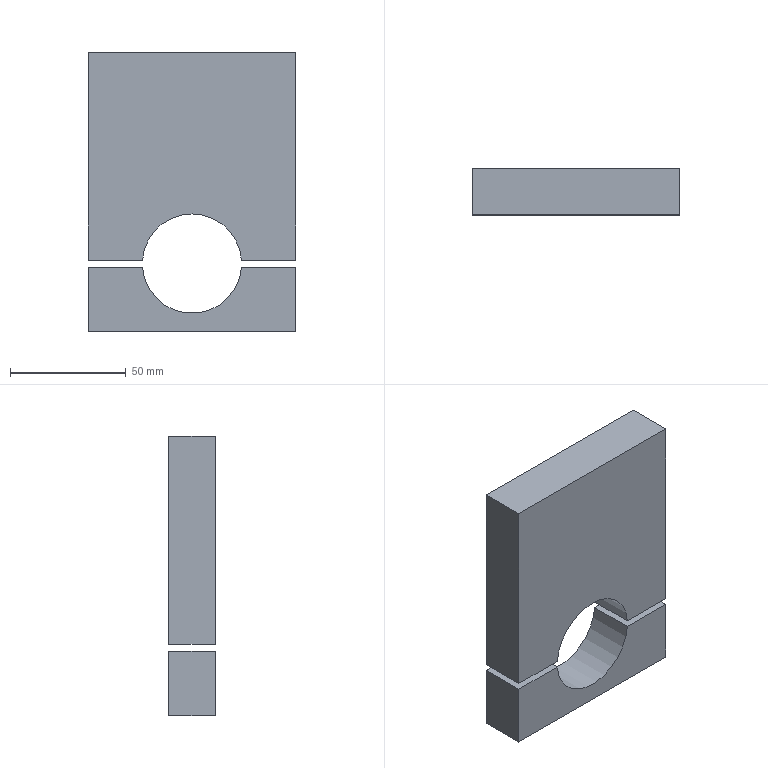Component | SolidWorks | YC1-250-04BalancerAssembly#16673-1_YC1-250-04-12#16673PipeSeat-1 | 2 solids | 29 faces | box 90 x 20 x 121 mm | volume 177905 mm3 | plane 14 | cylinder 11 | cone 4 | commonest cylinder face diameters 8.5 x4 11 x4 43 x3 | material Plain Carbon Steel
STEP:
#1=COLOUR_RGB('',0.7922,0.8196,0.9333);
#2=FILL_AREA_STYLE_COLOUR('',#1);
#3=FILL_AREA_STYLE('',(#2));
#4=SURFACE_STYLE_FILL_AREA(#3);
#5=SURFACE_SIDE_STYLE('',(#4));
#6=SURFACE_STYLE_USAGE(.BOTH.,#5);
#7=PRESENTATION_STYLE_ASSIGNMENT((#6));
#8=CARTESIAN_POINT('',(-16.929,179.528,-9.567));
#9=VERTEX_POINT('',#8);
#10=CARTESIAN_POINT('',(-16.496,179.528,-9.567));
#11=VERTEX_POINT('',#10);
#12=CARTESIAN_POINT('',(-16.713,179.528,-9.567));
#13=DIRECTION('',(0.,0.,1.));
#14=DIRECTION('',(-1.,0.,0.));
#15=AXIS2_PLACEMENT_3D('',#12,#13,#14);
#16=CIRCLE('',#15,0.2165);
#17=EDGE_CURVE('',#9,#11,#16,.T.);
#18=ORIENTED_EDGE('',*,*,#17,.T.);
#19=CARTESIAN_POINT('',(-16.496,179.528,-10.669));
#20=VERTEX_POINT('',#19);
#21=CARTESIAN_POINT('',(-16.496,179.528,-10.669));
#22=DIRECTION('',(0.,0.,-1.));
#23=VECTOR('',#22,39.37);
#24=LINE('',#21,#23);
#25=EDGE_CURVE('',#11,#20,#24,.T.);
#26=ORIENTED_EDGE('',*,*,#25,.T.);
#27=CARTESIAN_POINT('',(-16.929,179.528,-10.669));
#28=VERTEX_POINT('',#27);
#29=CARTESIAN_POINT('',(-16.713,179.528,-10.669));
#30=DIRECTION('',(0.,0.,-1.));
#31=DIRECTION('',(-1.,0.,0.));
#32=AXIS2_PLACEMENT_3D('',#29,#30,#31);
#33=CIRCLE('',#32,0.2165);
#34=EDGE_CURVE('',#20,#28,#33,.T.);
#35=ORIENTED_EDGE('',*,*,#34,.T.);
#36=CARTESIAN_POINT('',(-16.929,179.528,-10.669));
#37=DIRECTION('',(0.,0.,-1.));
#38=VECTOR('',#37,39.37);
#39=LINE('',#36,#38);
#40=EDGE_CURVE('',#9,#28,#39,.T.);
#41=ORIENTED_EDGE('',*,*,#40,.F.);
#42=EDGE_LOOP('',(#18,#26,#35,#41));
#43=FACE_OUTER_BOUND('',#42,.T.);
#44=CARTESIAN_POINT('',(-16.713,179.528,-10.669));
#45=DIRECTION('',(0.,0.,-1.));
#46=DIRECTION('',(-1.,0.,0.));
#47=AXIS2_PLACEMENT_3D('',#44,#45,#46);
#48=CYLINDRICAL_SURFACE('',#47,0.2165);
#49=ADVANCED_FACE('',(#43),#48,.F.);
#50=CARTESIAN_POINT('',(-19.724,179.528,-9.567));
#51=VERTEX_POINT('',#50);
#52=CARTESIAN_POINT('',(-19.291,179.528,-9.567));
#53=VERTEX_POINT('',#52);
#54=CARTESIAN_POINT('',(-19.508,179.528,-9.567));
#55=DIRECTION('',(0.,0.,1.));
#56=DIRECTION('',(-1.,0.,0.));
#57=AXIS2_PLACEMENT_3D('',#54,#55,#56);
#58=CIRCLE('',#57,0.2165);
#59=EDGE_CURVE('',#51,#53,#58,.T.);
#60=ORIENTED_EDGE('',*,*,#59,.T.);
#61=CARTESIAN_POINT('',(-19.291,179.528,-10.669));
#62=VERTEX_POINT('',#61);
#63=CARTESIAN_POINT('',(-19.291,179.528,-10.669));
#64=DIRECTION('',(0.,0.,-1.));
#65=VECTOR('',#64,39.37);
#66=LINE('',#63,#65);
#67=EDGE_CURVE('',#53,#62,#66,.T.);
#68=ORIENTED_EDGE('',*,*,#67,.T.);
#69=CARTESIAN_POINT('',(-19.724,179.528,-10.669));
#70=VERTEX_POINT('',#69);
#71=CARTESIAN_POINT('',(-19.508,179.528,-10.669));
#72=DIRECTION('',(0.,0.,-1.));
#73=DIRECTION('',(-1.,0.,0.));
#74=AXIS2_PLACEMENT_3D('',#71,#72,#73);
#75=CIRCLE('',#74,0.2165);
#76=EDGE_CURVE('',#62,#70,#75,.T.);
#77=ORIENTED_EDGE('',*,*,#76,.T.);
#78=CARTESIAN_POINT('',(-19.724,179.528,-10.669));
#79=DIRECTION('',(0.,0.,-1.));
#80=VECTOR('',#79,39.37);
#81=LINE('',#78,#80);
#82=EDGE_CURVE('',#51,#70,#81,.T.);
#83=ORIENTED_EDGE('',*,*,#82,.F.);
#84=EDGE_LOOP('',(#60,#68,#77,#83));
#85=FACE_OUTER_BOUND('',#84,.T.);
#86=CARTESIAN_POINT('',(-19.508,179.528,-10.669));
#87=DIRECTION('',(0.,0.,-1.));
#88=DIRECTION('',(-1.,0.,0.));
#89=AXIS2_PLACEMENT_3D('',#86,#87,#88);
#90=CYLINDRICAL_SURFACE('',#89,0.2165);
#91=ADVANCED_FACE('',(#85),#90,.F.);
#92=CARTESIAN_POINT('',(-19.882,179.134,-9.567));
#93=VERTEX_POINT('',#92);
#94=CARTESIAN_POINT('',(-19.882,179.134,-10.669));
#95=VERTEX_POINT('',#94);
#96=CARTESIAN_POINT('',(-19.882,179.134,-9.508));
#97=DIRECTION('',(0.,0.,-1.));
#98=VECTOR('',#97,39.37);
#99=LINE('',#96,#98);
#100=EDGE_CURVE('',#93,#95,#99,.T.);
#101=ORIENTED_EDGE('',*,*,#100,.T.);
#102=CARTESIAN_POINT('',(-16.339,179.134,-10.669));
#103=VERTEX_POINT('',#102);
#104=CARTESIAN_POINT('',(-18.11,179.134,-10.669));
#105=DIRECTION('',(1.,0.,0.));
#106=VECTOR('',#105,39.37);
#107=LINE('',#104,#106);
#108=EDGE_CURVE('',#95,#103,#107,.T.);
#109=ORIENTED_EDGE('',*,*,#108,.T.);
#110=CARTESIAN_POINT('',(-16.339,179.134,-9.567));
#111=VERTEX_POINT('',#110);
#112=CARTESIAN_POINT('',(-16.339,179.134,-9.508));
#113=DIRECTION('',(0.,0.,1.));
#114=VECTOR('',#113,39.37);
#115=LINE('',#112,#114);
#116=EDGE_CURVE('',#103,#111,#115,.T.);
#117=ORIENTED_EDGE('',*,*,#116,.T.);
#118=CARTESIAN_POINT('',(-17.266,179.134,-9.567));
#119=VERTEX_POINT('',#118);
#120=CARTESIAN_POINT('',(-18.11,179.134,-9.567));
#121=DIRECTION('',(-1.,0.,0.));
#122=VECTOR('',#121,39.37);
#123=LINE('',#120,#122);
#124=EDGE_CURVE('',#111,#119,#123,.T.);
#125=ORIENTED_EDGE('',*,*,#124,.T.);
#126=CARTESIAN_POINT('',(-18.955,179.134,-9.567));
#127=VERTEX_POINT('',#126);
#128=CARTESIAN_POINT('',(-18.11,179.134,-9.508));
#129=DIRECTION('',(0.,1.,0.));
#130=DIRECTION('',(0.,0.,1.));
#131=AXIS2_PLACEMENT_3D('',#128,#129,#130);
#132=CIRCLE('',#131,0.8465);
#133=EDGE_CURVE('',#119,#127,#132,.T.);
#134=ORIENTED_EDGE('',*,*,#133,.T.);
#135=CARTESIAN_POINT('',(-18.11,179.134,-9.567));
#136=DIRECTION('',(-1.,0.,0.));
#137=VECTOR('',#136,39.37);
#138=LINE('',#135,#137);
#139=EDGE_CURVE('',#127,#93,#138,.T.);
#140=ORIENTED_EDGE('',*,*,#139,.T.);
#141=EDGE_LOOP('',(#101,#109,#117,#125,#134,#140));
#142=FACE_OUTER_BOUND('',#141,.T.);
#143=CARTESIAN_POINT('',(-18.11,179.134,-9.508));
#144=DIRECTION('',(0.,-1.,0.));
#145=DIRECTION('',(0.,0.,-1.));
#146=AXIS2_PLACEMENT_3D('',#143,#144,#145);
#147=PLANE('',#146);
#148=ADVANCED_FACE('',(#142),#147,.T.);
#149=CARTESIAN_POINT('',(-16.339,179.921,-10.669));
#150=VERTEX_POINT('',#149);
#151=CARTESIAN_POINT('',(-16.339,179.134,-10.669));
#152=DIRECTION('',(0.,1.,0.));
#153=VECTOR('',#152,39.37);
#154=LINE('',#151,#153);
#155=EDGE_CURVE('',#103,#150,#154,.T.);
#156=ORIENTED_EDGE('',*,*,#155,.F.);
#157=ORIENTED_EDGE('',*,*,#108,.F.);
#158=CARTESIAN_POINT('',(-19.882,179.921,-10.669));
#159=VERTEX_POINT('',#158);
#160=CARTESIAN_POINT('',(-19.882,179.134,-10.669));
#161=DIRECTION('',(0.,-1.,0.));
#162=VECTOR('',#161,39.37);
#163=LINE('',#160,#162);
#164=EDGE_CURVE('',#159,#95,#163,.T.);
#165=ORIENTED_EDGE('',*,*,#164,.F.);
#166=CARTESIAN_POINT('',(-19.882,179.921,-10.669));
#167=DIRECTION('',(-1.,0.,-0.));
#168=VECTOR('',#167,39.37);
#169=LINE('',#166,#168);
#170=EDGE_CURVE('',#150,#159,#169,.T.);
#171=ORIENTED_EDGE('',*,*,#170,.F.);
#172=EDGE_LOOP('',(#156,#157,#165,#171));
#173=FACE_OUTER_BOUND('',#172,.T.);
#174=CARTESIAN_POINT('',(-16.713,179.528,-10.669));
#175=DIRECTION('',(0.,0.,-1.));
#176=DIRECTION('',(-1.,0.,0.));
#177=AXIS2_PLACEMENT_3D('',#174,#175,#176);
#178=CIRCLE('',#177,0.2165);
#179=EDGE_CURVE('',#28,#20,#178,.T.);
#180=ORIENTED_EDGE('',*,*,#179,.F.);
#181=ORIENTED_EDGE('',*,*,#34,.F.);
#182=EDGE_LOOP('',(#180,#181));
#183=FACE_BOUND('',#182,.T.);
#184=CARTESIAN_POINT('',(-19.508,179.528,-10.669));
#185=DIRECTION('',(0.,0.,-1.));
#186=DIRECTION('',(-1.,0.,0.));
#187=AXIS2_PLACEMENT_3D('',#184,#185,#186);
#188=CIRCLE('',#187,0.2165);
#189=EDGE_CURVE('',#70,#62,#188,.T.);
#190=ORIENTED_EDGE('',*,*,#189,.F.);
#191=ORIENTED_EDGE('',*,*,#76,.F.);
#192=EDGE_LOOP('',(#190,#191));
#193=FACE_BOUND('',#192,.T.);
#194=CARTESIAN_POINT('',(-19.882,179.134,-10.669));
#195=DIRECTION('',(-0.,0.,1.));
#196=DIRECTION('',(1.,0.,0.));
#197=AXIS2_PLACEMENT_3D('',#194,#195,#196);
#198=PLANE('',#197);
#199=ADVANCED_FACE('',(#173,#183,#193),#198,.F.);
#200=ORIENTED_EDGE('',*,*,#164,.T.);
#201=ORIENTED_EDGE('',*,*,#100,.F.);
#202=CARTESIAN_POINT('',(-19.882,179.921,-9.567));
#203=VERTEX_POINT('',#202);
#204=CARTESIAN_POINT('',(-19.882,179.134,-9.567));
#205=DIRECTION('',(0.,-1.,0.));
#206=VECTOR('',#205,39.37);
#207=LINE('',#204,#206);
#208=EDGE_CURVE('',#203,#93,#207,.T.);
#209=ORIENTED_EDGE('',*,*,#208,.F.);
#210=CARTESIAN_POINT('',(-19.882,179.921,-9.567));
#211=DIRECTION('',(-0.,0.,1.));
#212=VECTOR('',#211,39.37);
#213=LINE('',#210,#212);
#214=EDGE_CURVE('',#159,#203,#213,.T.);
#215=ORIENTED_EDGE('',*,*,#214,.F.);
#216=EDGE_LOOP('',(#200,#201,#209,#215));
#217=FACE_OUTER_BOUND('',#216,.T.);
#218=CARTESIAN_POINT('',(-19.882,179.134,-9.567));
#219=DIRECTION('',(1.,0.,0.));
#220=DIRECTION('',(0.,0.,-1.));
#221=AXIS2_PLACEMENT_3D('',#218,#219,#220);
#222=PLANE('',#221);
#223=ADVANCED_FACE('',(#217),#222,.F.);
#224=ORIENTED_EDGE('',*,*,#208,.T.);
#225=ORIENTED_EDGE('',*,*,#139,.F.);
#226=CARTESIAN_POINT('',(-18.955,179.921,-9.567));
#227=VERTEX_POINT('',#226);
#228=CARTESIAN_POINT('',(-18.955,179.134,-9.567));
#229=DIRECTION('',(0.,-1.,0.));
#230=VECTOR('',#229,39.37);
#231=LINE('',#228,#230);
#232=EDGE_CURVE('',#227,#127,#231,.T.);
#233=ORIENTED_EDGE('',*,*,#232,.F.);
#234=CARTESIAN_POINT('',(-19.882,179.921,-9.567));
#235=DIRECTION('',(1.,0.,0.));
#236=VECTOR('',#235,39.37);
#237=LINE('',#234,#236);
#238=EDGE_CURVE('',#203,#227,#237,.T.);
#239=ORIENTED_EDGE('',*,*,#238,.F.);
#240=EDGE_LOOP('',(#224,#225,#233,#239));
#241=FACE_OUTER_BOUND('',#240,.T.);
#242=ORIENTED_EDGE('',*,*,#59,.F.);
#243=CARTESIAN_POINT('',(-19.508,179.528,-9.567));
#244=DIRECTION('',(0.,0.,1.));
#245=DIRECTION('',(-1.,0.,0.));
#246=AXIS2_PLACEMENT_3D('',#243,#244,#245);
#247=CIRCLE('',#246,0.2165);
#248=EDGE_CURVE('',#53,#51,#247,.T.);
#249=ORIENTED_EDGE('',*,*,#248,.F.);
#250=EDGE_LOOP('',(#242,#249));
#251=FACE_BOUND('',#250,.T.);
#252=CARTESIAN_POINT('',(-19.882,179.134,-9.567));
#253=DIRECTION('',(0.,0.,-1.));
#254=DIRECTION('',(-1.,0.,-0.));
#255=AXIS2_PLACEMENT_3D('',#252,#253,#254);
#256=PLANE('',#255);
#257=ADVANCED_FACE('',(#241,#251),#256,.F.);
#258=ORIENTED_EDGE('',*,*,#232,.T.);
#259=ORIENTED_EDGE('',*,*,#133,.F.);
#260=CARTESIAN_POINT('',(-17.266,179.921,-9.567));
#261=VERTEX_POINT('',#260);
#262=CARTESIAN_POINT('',(-17.266,179.134,-9.567));
#263=DIRECTION('',(0.,-1.,0.));
#264=VECTOR('',#263,39.37);
#265=LINE('',#262,#264);
#266=EDGE_CURVE('',#261,#119,#265,.T.);
#267=ORIENTED_EDGE('',*,*,#266,.F.);
#268=CARTESIAN_POINT('',(-18.11,179.921,-9.508));
#269=DIRECTION('',(0.,-1.,0.));
#270=DIRECTION('',(0.,0.,1.));
#271=AXIS2_PLACEMENT_3D('',#268,#269,#270);
#272=CIRCLE('',#271,0.8465);
#273=EDGE_CURVE('',#227,#261,#272,.T.);
#274=ORIENTED_EDGE('',*,*,#273,.F.);
#275=EDGE_LOOP('',(#258,#259,#267,#274));
#276=FACE_OUTER_BOUND('',#275,.T.);
#277=CARTESIAN_POINT('',(-18.11,179.134,-9.508));
#278=DIRECTION('',(0.,1.,0.));
#279=DIRECTION('',(0.,0.,1.));
#280=AXIS2_PLACEMENT_3D('',#277,#278,#279);
#281=CYLINDRICAL_SURFACE('',#280,0.8465);
#282=ADVANCED_FACE('',(#276),#281,.F.);
#283=ORIENTED_EDGE('',*,*,#266,.T.);
#284=ORIENTED_EDGE('',*,*,#124,.F.);
#285=CARTESIAN_POINT('',(-16.339,179.921,-9.567));
#286=VERTEX_POINT('',#285);
#287=CARTESIAN_POINT('',(-16.339,179.134,-9.567));
#288=DIRECTION('',(0.,-1.,0.));
#289=VECTOR('',#288,39.37);
#290=LINE('',#287,#289);
#291=EDGE_CURVE('',#286,#111,#290,.T.);
#292=ORIENTED_EDGE('',*,*,#291,.F.);
#293=CARTESIAN_POINT('',(-17.266,179.921,-9.567));
#294=DIRECTION('',(1.,0.,0.));
#295=VECTOR('',#294,39.37);
#296=LINE('',#293,#295);
#297=EDGE_CURVE('',#261,#286,#296,.T.);
#298=ORIENTED_EDGE('',*,*,#297,.F.);
#299=EDGE_LOOP('',(#283,#284,#292,#298));
#300=FACE_OUTER_BOUND('',#299,.T.);
#301=ORIENTED_EDGE('',*,*,#17,.F.);
#302=CARTESIAN_POINT('',(-16.713,179.528,-9.567));
#303=DIRECTION('',(0.,0.,1.));
#304=DIRECTION('',(-1.,0.,0.));
#305=AXIS2_PLACEMENT_3D('',#302,#303,#304);
#306=CIRCLE('',#305,0.2165);
#307=EDGE_CURVE('',#11,#9,#306,.T.);
#308=ORIENTED_EDGE('',*,*,#307,.F.);
#309=EDGE_LOOP('',(#301,#308));
#310=FACE_BOUND('',#309,.T.);
#311=CARTESIAN_POINT('',(-17.266,179.134,-9.567));
#312=DIRECTION('',(0.,0.,-1.));
#313=DIRECTION('',(-1.,0.,-0.));
#314=AXIS2_PLACEMENT_3D('',#311,#312,#313);
#315=PLANE('',#314);
#316=ADVANCED_FACE('',(#300,#310),#315,.F.);
#317=ORIENTED_EDGE('',*,*,#291,.T.);
#318=ORIENTED_EDGE('',*,*,#116,.F.);
#319=ORIENTED_EDGE('',*,*,#155,.T.);
#320=CARTESIAN_POINT('',(-16.339,179.921,-9.567));
#321=DIRECTION('',(-0.,0.,-1.));
#322=VECTOR('',#321,39.37);
#323=LINE('',#320,#322);
#324=EDGE_CURVE('',#286,#150,#323,.T.);
#325=ORIENTED_EDGE('',*,*,#324,.F.);
#326=EDGE_LOOP('',(#317,#318,#319,#325));
#327=FACE_OUTER_BOUND('',#326,.T.);
#328=CARTESIAN_POINT('',(-16.339,179.134,-9.567));
#329=DIRECTION('',(-1.,0.,0.));
#330=DIRECTION('',(0.,0.,1.));
#331=AXIS2_PLACEMENT_3D('',#328,#329,#330);
#332=PLANE('',#331);
#333=ADVANCED_FACE('',(#327),#332,.F.);
#334=ORIENTED_EDGE('',*,*,#170,.T.);
#335=ORIENTED_EDGE('',*,*,#214,.T.);
#336=ORIENTED_EDGE('',*,*,#238,.T.);
#337=ORIENTED_EDGE('',*,*,#273,.T.);
#338=ORIENTED_EDGE('',*,*,#297,.T.);
#339=ORIENTED_EDGE('',*,*,#324,.T.);
#340=EDGE_LOOP('',(#334,#335,#336,#337,#338,#339));
#341=FACE_OUTER_BOUND('',#340,.T.);
#342=CARTESIAN_POINT('',(-18.11,179.921,-9.508));
#343=DIRECTION('',(0.,-1.,0.));
#344=DIRECTION('',(0.,0.,-1.));
#345=AXIS2_PLACEMENT_3D('',#342,#343,#344);
#346=PLANE('',#345);
#347=ADVANCED_FACE('',(#341),#346,.F.);
#348=ORIENTED_EDGE('',*,*,#25,.F.);
#349=ORIENTED_EDGE('',*,*,#307,.T.);
#350=ORIENTED_EDGE('',*,*,#40,.T.);
#351=ORIENTED_EDGE('',*,*,#179,.T.);
#352=EDGE_LOOP('',(#348,#349,#350,#351));
#353=FACE_OUTER_BOUND('',#352,.T.);
#354=CARTESIAN_POINT('',(-16.713,179.528,-10.669));
#355=DIRECTION('',(0.,0.,-1.));
#356=DIRECTION('',(-1.,0.,0.));
#357=AXIS2_PLACEMENT_3D('',#354,#355,#356);
#358=CYLINDRICAL_SURFACE('',#357,0.2165);
#359=ADVANCED_FACE('',(#353),#358,.F.);
#360=ORIENTED_EDGE('',*,*,#67,.F.);
#361=ORIENTED_EDGE('',*,*,#248,.T.);
#362=ORIENTED_EDGE('',*,*,#82,.T.);
#363=ORIENTED_EDGE('',*,*,#189,.T.);
#364=EDGE_LOOP('',(#360,#361,#362,#363));
#365=FACE_OUTER_BOUND('',#364,.T.);
#366=CARTESIAN_POINT('',(-19.508,179.528,-10.669));
#367=DIRECTION('',(0.,0.,-1.));
#368=DIRECTION('',(-1.,0.,0.));
#369=AXIS2_PLACEMENT_3D('',#366,#367,#368);
#370=CYLINDRICAL_SURFACE('',#369,0.2165);
#371=ADVANCED_FACE('',(#365),#370,.F.);
#372=CLOSED_SHELL('',(#49,#91,#148,#199,#223,#257,#282,#316,#333,#347,#359,#371));
#373=MANIFOLD_SOLID_BREP('',#372);
#374=STYLED_ITEM('',(#7),#373);
#375=PRESENTATION_LAYER_ASSIGNMENT('','',(#374));
#376=COLOUR_RGB('',0.7922,0.8196,0.9333);
#377=FILL_AREA_STYLE_COLOUR('',#376);
#378=FILL_AREA_STYLE('',(#377));
#379=SURFACE_STYLE_FILL_AREA(#378);
#380=SURFACE_SIDE_STYLE('',(#379));
#381=SURFACE_STYLE_USAGE(.BOTH.,#380);
#382=PRESENTATION_STYLE_ASSIGNMENT((#381));
#383=CARTESIAN_POINT('',(-18.11,179.134,-8.661));
#384=VERTEX_POINT('',#383);
#385=CARTESIAN_POINT('',(-17.266,179.134,-9.449));
#386=VERTEX_POINT('',#385);
#387=CARTESIAN_POINT('',(-18.11,179.134,-9.508));
#388=DIRECTION('',(0.,1.,0.));
#389=DIRECTION('',(0.,0.,1.));
#390=AXIS2_PLACEMENT_3D('',#387,#388,#389);
#391=CIRCLE('',#390,0.8465);
#392=EDGE_CURVE('',#384,#386,#391,.T.);
#393=ORIENTED_EDGE('',*,*,#392,.F.);
#394=CARTESIAN_POINT('',(-18.11,179.921,-8.661));
#395=VERTEX_POINT('',#394);
#396=CARTESIAN_POINT('',(-18.11,179.134,-8.661));
#397=DIRECTION('',(0.,1.,0.));
#398=VECTOR('',#397,39.37);
#399=LINE('',#396,#398);
#400=EDGE_CURVE('',#384,#395,#399,.T.);
#401=ORIENTED_EDGE('',*,*,#400,.T.);
#402=CARTESIAN_POINT('',(-17.266,179.921,-9.449));
#403=VERTEX_POINT('',#402);
#404=CARTESIAN_POINT('',(-18.11,179.921,-9.508));
#405=DIRECTION('',(0.,-1.,0.));
#406=DIRECTION('',(0.,0.,1.));
#407=AXIS2_PLACEMENT_3D('',#404,#405,#406);
#408=CIRCLE('',#407,0.8465);
#409=EDGE_CURVE('',#403,#395,#408,.T.);
#410=ORIENTED_EDGE('',*,*,#409,.F.);
#411=CARTESIAN_POINT('',(-17.266,179.134,-9.449));
#412=DIRECTION('',(0.,-1.,0.));
#413=VECTOR('',#412,39.37);
#414=LINE('',#411,#413);
#415=EDGE_CURVE('',#403,#386,#414,.T.);
#416=ORIENTED_EDGE('',*,*,#415,.T.);
#417=EDGE_LOOP('',(#393,#401,#410,#416));
#418=FACE_OUTER_BOUND('',#417,.T.);
#419=CARTESIAN_POINT('',(-18.11,179.134,-9.508));
#420=DIRECTION('',(0.,1.,0.));
#421=DIRECTION('',(0.,0.,1.));
#422=AXIS2_PLACEMENT_3D('',#419,#420,#421);
#423=CYLINDRICAL_SURFACE('',#422,0.8465);
#424=ADVANCED_FACE('',(#418),#423,.F.);
#425=CARTESIAN_POINT('',(-16.545,179.528,-8.543));
#426=VERTEX_POINT('',#425);
#427=CARTESIAN_POINT('',(-16.713,179.36,-8.543));
#428=VERTEX_POINT('',#427);
#429=CARTESIAN_POINT('',(-16.713,179.528,-8.543));
#430=DIRECTION('',(0.,0.,-1.));
#431=DIRECTION('',(-1.,0.,0.));
#432=AXIS2_PLACEMENT_3D('',#429,#430,#431);
#433=CIRCLE('',#432,0.1673);
#434=EDGE_CURVE('',#426,#428,#433,.T.);
#435=ORIENTED_EDGE('',*,*,#434,.F.);
#436=CARTESIAN_POINT('',(-16.545,179.528,-9.449));
#437=VERTEX_POINT('',#436);
#438=CARTESIAN_POINT('',(-16.545,179.528,-9.449));
#439=DIRECTION('',(0.,0.,-1.));
#440=VECTOR('',#439,39.37);
#441=LINE('',#438,#440);
#442=EDGE_CURVE('',#426,#437,#441,.T.);
#443=ORIENTED_EDGE('',*,*,#442,.T.);
#444=CARTESIAN_POINT('',(-16.88,179.528,-9.449));
#445=VERTEX_POINT('',#444);
#446=CARTESIAN_POINT('',(-16.713,179.528,-9.449));
#447=DIRECTION('',(0.,0.,-1.));
#448=DIRECTION('',(-1.,0.,0.));
#449=AXIS2_PLACEMENT_3D('',#446,#447,#448);
#450=CIRCLE('',#449,0.1673);
#451=EDGE_CURVE('',#437,#445,#450,.T.);
#452=ORIENTED_EDGE('',*,*,#451,.T.);
#453=CARTESIAN_POINT('',(-16.88,179.528,-8.543));
#454=VERTEX_POINT('',#453);
#455=CARTESIAN_POINT('',(-16.88,179.528,-9.449));
#456=DIRECTION('',(0.,0.,-1.));
#457=VECTOR('',#456,39.37);
#458=LINE('',#455,#457);
#459=EDGE_CURVE('',#454,#445,#458,.T.);
#460=ORIENTED_EDGE('',*,*,#459,.F.);
#461=CARTESIAN_POINT('',(-16.713,179.528,-8.543));
#462=DIRECTION('',(0.,0.,-1.));
#463=DIRECTION('',(-1.,0.,0.));
#464=AXIS2_PLACEMENT_3D('',#461,#462,#463);
#465=CIRCLE('',#464,0.1673);
#466=EDGE_CURVE('',#428,#454,#465,.T.);
#467=ORIENTED_EDGE('',*,*,#466,.F.);
#468=EDGE_LOOP('',(#435,#443,#452,#460,#467));
#469=FACE_OUTER_BOUND('',#468,.T.);
#470=CARTESIAN_POINT('',(-16.713,179.528,-9.449));
#471=DIRECTION('',(0.,0.,-1.));
#472=DIRECTION('',(-1.,0.,0.));
#473=AXIS2_PLACEMENT_3D('',#470,#471,#472);
#474=CYLINDRICAL_SURFACE('',#473,0.1673);
#475=ADVANCED_FACE('',(#469),#474,.F.);
#476=CARTESIAN_POINT('',(-19.341,179.528,-8.543));
#477=VERTEX_POINT('',#476);
#478=CARTESIAN_POINT('',(-19.675,179.528,-8.543));
#479=VERTEX_POINT('',#478);
#480=CARTESIAN_POINT('',(-19.508,179.528,-8.543));
#481=DIRECTION('',(0.,0.,-1.));
#482=DIRECTION('',(-1.,0.,0.));
#483=AXIS2_PLACEMENT_3D('',#480,#481,#482);
#484=CIRCLE('',#483,0.1673);
#485=EDGE_CURVE('',#477,#479,#484,.T.);
#486=ORIENTED_EDGE('',*,*,#485,.F.);
#487=CARTESIAN_POINT('',(-19.341,179.528,-9.449));
#488=VERTEX_POINT('',#487);
#489=CARTESIAN_POINT('',(-19.341,179.528,-9.449));
#490=DIRECTION('',(0.,0.,-1.));
#491=VECTOR('',#490,39.37);
#492=LINE('',#489,#491);
#493=EDGE_CURVE('',#477,#488,#492,.T.);
#494=ORIENTED_EDGE('',*,*,#493,.T.);
#495=CARTESIAN_POINT('',(-19.675,179.528,-9.449));
#496=VERTEX_POINT('',#495);
#497=CARTESIAN_POINT('',(-19.508,179.528,-9.449));
#498=DIRECTION('',(0.,0.,-1.));
#499=DIRECTION('',(-1.,0.,0.));
#500=AXIS2_PLACEMENT_3D('',#497,#498,#499);
#501=CIRCLE('',#500,0.1673);
#502=EDGE_CURVE('',#488,#496,#501,.T.);
#503=ORIENTED_EDGE('',*,*,#502,.T.);
#504=CARTESIAN_POINT('',(-19.675,179.528,-9.449));
#505=DIRECTION('',(0.,0.,-1.));
#506=VECTOR('',#505,39.37);
#507=LINE('',#504,#506);
#508=EDGE_CURVE('',#479,#496,#507,.T.);
#509=ORIENTED_EDGE('',*,*,#508,.F.);
#510=EDGE_LOOP('',(#486,#494,#503,#509));
#511=FACE_OUTER_BOUND('',#510,.T.);
#512=CARTESIAN_POINT('',(-19.508,179.528,-9.449));
#513=DIRECTION('',(0.,0.,-1.));
#514=DIRECTION('',(-1.,0.,0.));
#515=AXIS2_PLACEMENT_3D('',#512,#513,#514);
#516=CYLINDRICAL_SURFACE('',#515,0.1673);
#517=ADVANCED_FACE('',(#511),#516,.F.);
#518=CARTESIAN_POINT('',(-16.713,179.528,-8.443));
#519=VERTEX_POINT('',#518);
#520=CARTESIAN_POINT('',(-16.713,179.695,-8.543));
#521=VERTEX_POINT('',#520);
#522=CARTESIAN_POINT('',(-16.713,179.695,-8.543));
#523=DIRECTION('',(0.,0.8572,-0.515));
#524=VECTOR('',#523,39.37);
#525=LINE('',#522,#524);
#526=EDGE_CURVE('',#519,#521,#525,.T.);
#527=ORIENTED_EDGE('',*,*,#526,.F.);
#528=CARTESIAN_POINT('',(-16.713,179.36,-8.543));
#529=DIRECTION('',(0.,-0.8572,-0.515));
#530=VECTOR('',#529,39.37);
#531=LINE('',#528,#530);
#532=EDGE_CURVE('',#519,#428,#531,.T.);
#533=ORIENTED_EDGE('',*,*,#532,.T.);
#534=ORIENTED_EDGE('',*,*,#466,.T.);
#535=CARTESIAN_POINT('',(-16.713,179.528,-8.543));
#536=DIRECTION('',(0.,0.,-1.));
#537=DIRECTION('',(-1.,0.,0.));
#538=AXIS2_PLACEMENT_3D('',#535,#536,#537);
#539=CIRCLE('',#538,0.1673);
#540=EDGE_CURVE('',#454,#521,#539,.T.);
#541=ORIENTED_EDGE('',*,*,#540,.T.);
#542=EDGE_LOOP('',(#527,#533,#534,#541));
#543=FACE_OUTER_BOUND('',#542,.T.);
#544=CARTESIAN_POINT('',(-16.713,179.528,-8.543));
#545=DIRECTION('',(0.,-0.,-1.));
#546=DIRECTION('',(0.,1.,0.));
#547=AXIS2_PLACEMENT_3D('',#544,#545,#546);
#548=CONICAL_SURFACE('',#547,0.1673,1.03);
#549=ADVANCED_FACE('',(#543),#548,.F.);
#550=CARTESIAN_POINT('',(-19.508,179.528,-8.443));
#551=VERTEX_POINT('',#550);
#552=CARTESIAN_POINT('',(-19.675,179.528,-8.543));
#553=DIRECTION('',(-0.8572,0.,-0.515));
#554=VECTOR('',#553,39.37);
#555=LINE('',#552,#554);
#556=EDGE_CURVE('',#551,#479,#555,.T.);
#557=ORIENTED_EDGE('',*,*,#556,.F.);
#558=CARTESIAN_POINT('',(-19.341,179.528,-8.543));
#559=DIRECTION('',(0.8572,0.,-0.515));
#560=VECTOR('',#559,39.37);
#561=LINE('',#558,#560);
#562=EDGE_CURVE('',#551,#477,#561,.T.);
#563=ORIENTED_EDGE('',*,*,#562,.T.);
#564=ORIENTED_EDGE('',*,*,#485,.T.);
#565=EDGE_LOOP('',(#557,#563,#564));
#566=FACE_OUTER_BOUND('',#565,.T.);
#567=CARTESIAN_POINT('',(-19.508,179.528,-8.543));
#568=DIRECTION('',(0.,0.,-1.));
#569=DIRECTION('',(-1.,0.,0.));
#570=AXIS2_PLACEMENT_3D('',#567,#568,#569);
#571=CONICAL_SURFACE('',#570,0.1673,1.03);
#572=ADVANCED_FACE('',(#566),#571,.F.);
#573=CARTESIAN_POINT('',(-16.339,179.134,-9.449));
#574=VERTEX_POINT('',#573);
#575=CARTESIAN_POINT('',(-16.339,179.134,-5.906));
#576=VERTEX_POINT('',#575);
#577=CARTESIAN_POINT('',(-16.339,179.134,-9.508));
#578=DIRECTION('',(0.,0.,1.));
#579=VECTOR('',#578,39.37);
#580=LINE('',#577,#579);
#581=EDGE_CURVE('',#574,#576,#580,.T.);
#582=ORIENTED_EDGE('',*,*,#581,.T.);
#583=CARTESIAN_POINT('',(-19.882,179.134,-5.906));
#584=VERTEX_POINT('',#583);
#585=CARTESIAN_POINT('',(-18.11,179.134,-5.906));
#586=DIRECTION('',(-1.,0.,0.));
#587=VECTOR('',#586,39.37);
#588=LINE('',#585,#587);
#589=EDGE_CURVE('',#576,#584,#588,.T.);
#590=ORIENTED_EDGE('',*,*,#589,.T.);
#591=CARTESIAN_POINT('',(-19.882,179.134,-9.449));
#592=VERTEX_POINT('',#591);
#593=CARTESIAN_POINT('',(-19.882,179.134,-9.508));
#594=DIRECTION('',(0.,0.,-1.));
#595=VECTOR('',#594,39.37);
#596=LINE('',#593,#595);
#597=EDGE_CURVE('',#584,#592,#596,.T.);
#598=ORIENTED_EDGE('',*,*,#597,.T.);
#599=CARTESIAN_POINT('',(-18.955,179.134,-9.449));
#600=VERTEX_POINT('',#599);
#601=CARTESIAN_POINT('',(-18.11,179.134,-9.449));
#602=DIRECTION('',(1.,0.,0.));
#603=VECTOR('',#602,39.37);
#604=LINE('',#601,#603);
#605=EDGE_CURVE('',#592,#600,#604,.T.);
#606=ORIENTED_EDGE('',*,*,#605,.T.);
#607=CARTESIAN_POINT('',(-18.11,179.134,-9.508));
#608=DIRECTION('',(0.,1.,0.));
#609=DIRECTION('',(0.,0.,1.));
#610=AXIS2_PLACEMENT_3D('',#607,#608,#609);
#611=CIRCLE('',#610,0.8465);
#612=EDGE_CURVE('',#600,#384,#611,.T.);
#613=ORIENTED_EDGE('',*,*,#612,.T.);
#614=ORIENTED_EDGE('',*,*,#392,.T.);
#615=CARTESIAN_POINT('',(-18.11,179.134,-9.449));
#616=DIRECTION('',(1.,0.,0.));
#617=VECTOR('',#616,39.37);
#618=LINE('',#615,#617);
#619=EDGE_CURVE('',#386,#574,#618,.T.);
#620=ORIENTED_EDGE('',*,*,#619,.T.);
#621=EDGE_LOOP('',(#582,#590,#598,#606,#613,#614,#620));
#622=FACE_OUTER_BOUND('',#621,.T.);
#623=CARTESIAN_POINT('',(-18.11,179.134,-9.508));
#624=DIRECTION('',(0.,-1.,0.));
#625=DIRECTION('',(0.,0.,-1.));
#626=AXIS2_PLACEMENT_3D('',#623,#624,#625);
#627=PLANE('',#626);
#628=ADVANCED_FACE('',(#622),#627,.T.);
#629=CARTESIAN_POINT('',(-19.882,179.921,-5.906));
#630=VERTEX_POINT('',#629);
#631=CARTESIAN_POINT('',(-19.882,179.134,-5.906));
#632=DIRECTION('',(0.,1.,0.));
#633=VECTOR('',#632,39.37);
#634=LINE('',#631,#633);
#635=EDGE_CURVE('',#584,#630,#634,.T.);
#636=ORIENTED_EDGE('',*,*,#635,.F.);
#637=ORIENTED_EDGE('',*,*,#589,.F.);
#638=CARTESIAN_POINT('',(-16.339,179.921,-5.906));
#639=VERTEX_POINT('',#638);
#640=CARTESIAN_POINT('',(-16.339,179.134,-5.906));
#641=DIRECTION('',(0.,-1.,0.));
#642=VECTOR('',#641,39.37);
#643=LINE('',#640,#642);
#644=EDGE_CURVE('',#639,#576,#643,.T.);
#645=ORIENTED_EDGE('',*,*,#644,.F.);
#646=CARTESIAN_POINT('',(-19.882,179.921,-5.906));
#647=DIRECTION('',(1.,0.,0.));
#648=VECTOR('',#647,39.37);
#649=LINE('',#646,#648);
#650=EDGE_CURVE('',#630,#639,#649,.T.);
#651=ORIENTED_EDGE('',*,*,#650,.F.);
#652=EDGE_LOOP('',(#636,#637,#645,#651));
#653=FACE_OUTER_BOUND('',#652,.T.);
#654=CARTESIAN_POINT('',(-19.882,179.134,-5.906));
#655=DIRECTION('',(0.,0.,-1.));
#656=DIRECTION('',(-1.,0.,-0.));
#657=AXIS2_PLACEMENT_3D('',#654,#655,#656);
#658=PLANE('',#657);
#659=ADVANCED_FACE('',(#653),#658,.F.);
#660=ORIENTED_EDGE('',*,*,#644,.T.);
#661=ORIENTED_EDGE('',*,*,#581,.F.);
#662=CARTESIAN_POINT('',(-16.339,179.921,-9.449));
#663=VERTEX_POINT('',#662);
#664=CARTESIAN_POINT('',(-16.339,179.134,-9.449));
#665=DIRECTION('',(0.,-1.,0.));
#666=VECTOR('',#665,39.37);
#667=LINE('',#664,#666);
#668=EDGE_CURVE('',#663,#574,#667,.T.);
#669=ORIENTED_EDGE('',*,*,#668,.F.);
#670=CARTESIAN_POINT('',(-16.339,179.921,-5.906));
#671=DIRECTION('',(0.,0.,-1.));
#672=VECTOR('',#671,39.37);
#673=LINE('',#670,#672);
#674=EDGE_CURVE('',#639,#663,#673,.T.);
#675=ORIENTED_EDGE('',*,*,#674,.F.);
#676=EDGE_LOOP('',(#660,#661,#669,#675));
#677=FACE_OUTER_BOUND('',#676,.T.);
#678=CARTESIAN_POINT('',(-16.339,179.134,-5.906));
#679=DIRECTION('',(-1.,0.,-0.));
#680=DIRECTION('',(-0.,0.,1.));
#681=AXIS2_PLACEMENT_3D('',#678,#679,#680);
#682=PLANE('',#681);
#683=ADVANCED_FACE('',(#677),#682,.F.);
#684=ORIENTED_EDGE('',*,*,#668,.T.);
#685=ORIENTED_EDGE('',*,*,#619,.F.);
#686=ORIENTED_EDGE('',*,*,#415,.F.);
#687=CARTESIAN_POINT('',(-17.266,179.921,-9.449));
#688=DIRECTION('',(-1.,0.,-0.));
#689=VECTOR('',#688,39.37);
#690=LINE('',#687,#689);
#691=EDGE_CURVE('',#663,#403,#690,.T.);
#692=ORIENTED_EDGE('',*,*,#691,.F.);
#693=EDGE_LOOP('',(#684,#685,#686,#692));
#694=FACE_OUTER_BOUND('',#693,.T.);
#695=CARTESIAN_POINT('',(-16.713,179.528,-9.449));
#696=DIRECTION('',(0.,0.,-1.));
#697=DIRECTION('',(-1.,0.,0.));
#698=AXIS2_PLACEMENT_3D('',#695,#696,#697);
#699=CIRCLE('',#698,0.1673);
#700=EDGE_CURVE('',#445,#437,#699,.T.);
#701=ORIENTED_EDGE('',*,*,#700,.F.);
#702=ORIENTED_EDGE('',*,*,#451,.F.);
#703=EDGE_LOOP('',(#701,#702));
#704=FACE_BOUND('',#703,.T.);
#705=CARTESIAN_POINT('',(-17.266,179.134,-9.449));
#706=DIRECTION('',(-0.,0.,1.));
#707=DIRECTION('',(1.,0.,0.));
#708=AXIS2_PLACEMENT_3D('',#705,#706,#707);
#709=PLANE('',#708);
#710=ADVANCED_FACE('',(#694,#704),#709,.F.);
#711=ORIENTED_EDGE('',*,*,#400,.F.);
#712=ORIENTED_EDGE('',*,*,#612,.F.);
#713=CARTESIAN_POINT('',(-18.955,179.921,-9.449));
#714=VERTEX_POINT('',#713);
#715=CARTESIAN_POINT('',(-18.955,179.134,-9.449));
#716=DIRECTION('',(0.,-1.,0.));
#717=VECTOR('',#716,39.37);
#718=LINE('',#715,#717);
#719=EDGE_CURVE('',#714,#600,#718,.T.);
#720=ORIENTED_EDGE('',*,*,#719,.F.);
#721=CARTESIAN_POINT('',(-18.11,179.921,-9.508));
#722=DIRECTION('',(0.,-1.,0.));
#723=DIRECTION('',(0.,0.,1.));
#724=AXIS2_PLACEMENT_3D('',#721,#722,#723);
#725=CIRCLE('',#724,0.8465);
#726=EDGE_CURVE('',#395,#714,#725,.T.);
#727=ORIENTED_EDGE('',*,*,#726,.F.);
#728=EDGE_LOOP('',(#711,#712,#720,#727));
#729=FACE_OUTER_BOUND('',#728,.T.);
#730=CARTESIAN_POINT('',(-18.11,179.134,-9.508));
#731=DIRECTION('',(0.,1.,0.));
#732=DIRECTION('',(0.,0.,1.));
#733=AXIS2_PLACEMENT_3D('',#730,#731,#732);
#734=CYLINDRICAL_SURFACE('',#733,0.8465);
#735=ADVANCED_FACE('',(#729),#734,.F.);
#736=ORIENTED_EDGE('',*,*,#719,.T.);
#737=ORIENTED_EDGE('',*,*,#605,.F.);
#738=CARTESIAN_POINT('',(-19.882,179.921,-9.449));
#739=VERTEX_POINT('',#738);
#740=CARTESIAN_POINT('',(-19.882,179.134,-9.449));
#741=DIRECTION('',(0.,-1.,0.));
#742=VECTOR('',#741,39.37);
#743=LINE('',#740,#742);
#744=EDGE_CURVE('',#739,#592,#743,.T.);
#745=ORIENTED_EDGE('',*,*,#744,.F.);
#746=CARTESIAN_POINT('',(-19.882,179.921,-9.449));
#747=DIRECTION('',(-1.,0.,0.));
#748=VECTOR('',#747,39.37);
#749=LINE('',#746,#748);
#750=EDGE_CURVE('',#714,#739,#749,.T.);
#751=ORIENTED_EDGE('',*,*,#750,.F.);
#752=EDGE_LOOP('',(#736,#737,#745,#751));
#753=FACE_OUTER_BOUND('',#752,.T.);
#754=CARTESIAN_POINT('',(-19.508,179.528,-9.449));
#755=DIRECTION('',(0.,0.,-1.));
#756=DIRECTION('',(-1.,0.,0.));
#757=AXIS2_PLACEMENT_3D('',#754,#755,#756);
#758=CIRCLE('',#757,0.1673);
#759=EDGE_CURVE('',#496,#488,#758,.T.);
#760=ORIENTED_EDGE('',*,*,#759,.F.);
#761=ORIENTED_EDGE('',*,*,#502,.F.);
#762=EDGE_LOOP('',(#760,#761));
#763=FACE_BOUND('',#762,.T.);
#764=CARTESIAN_POINT('',(-19.882,179.134,-9.449));
#765=DIRECTION('',(0.,0.,1.));
#766=DIRECTION('',(1.,0.,-0.));
#767=AXIS2_PLACEMENT_3D('',#764,#765,#766);
#768=PLANE('',#767);
#769=ADVANCED_FACE('',(#753,#763),#768,.F.);
#770=ORIENTED_EDGE('',*,*,#744,.T.);
#771=ORIENTED_EDGE('',*,*,#597,.F.);
#772=ORIENTED_EDGE('',*,*,#635,.T.);
#773=CARTESIAN_POINT('',(-19.882,179.921,-5.906));
#774=DIRECTION('',(-0.,0.,1.));
#775=VECTOR('',#774,39.37);
#776=LINE('',#773,#775);
#777=EDGE_CURVE('',#739,#630,#776,.T.);
#778=ORIENTED_EDGE('',*,*,#777,.F.);
#779=EDGE_LOOP('',(#770,#771,#772,#778));
#780=FACE_OUTER_BOUND('',#779,.T.);
#781=CARTESIAN_POINT('',(-19.882,179.134,-5.906));
#782=DIRECTION('',(1.,0.,0.));
#783=DIRECTION('',(0.,0.,-1.));
#784=AXIS2_PLACEMENT_3D('',#781,#782,#783);
#785=PLANE('',#784);
#786=ADVANCED_FACE('',(#780),#785,.F.);
#787=ORIENTED_EDGE('',*,*,#650,.T.);
#788=ORIENTED_EDGE('',*,*,#674,.T.);
#789=ORIENTED_EDGE('',*,*,#691,.T.);
#790=ORIENTED_EDGE('',*,*,#409,.T.);
#791=ORIENTED_EDGE('',*,*,#726,.T.);
#792=ORIENTED_EDGE('',*,*,#750,.T.);
#793=ORIENTED_EDGE('',*,*,#777,.T.);
#794=EDGE_LOOP('',(#787,#788,#789,#790,#791,#792,#793));
#795=FACE_OUTER_BOUND('',#794,.T.);
#796=CARTESIAN_POINT('',(-18.11,179.921,-9.508));
#797=DIRECTION('',(0.,-1.,0.));
#798=DIRECTION('',(0.,0.,-1.));
#799=AXIS2_PLACEMENT_3D('',#796,#797,#798);
#800=PLANE('',#799);
#801=ADVANCED_FACE('',(#795),#800,.F.);
#802=ORIENTED_EDGE('',*,*,#442,.F.);
#803=CARTESIAN_POINT('',(-16.713,179.528,-8.543));
#804=DIRECTION('',(0.,0.,-1.));
#805=DIRECTION('',(-1.,0.,0.));
#806=AXIS2_PLACEMENT_3D('',#803,#804,#805);
#807=CIRCLE('',#806,0.1673);
#808=EDGE_CURVE('',#521,#426,#807,.T.);
#809=ORIENTED_EDGE('',*,*,#808,.F.);
#810=ORIENTED_EDGE('',*,*,#540,.F.);
#811=ORIENTED_EDGE('',*,*,#459,.T.);
#812=ORIENTED_EDGE('',*,*,#700,.T.);
#813=EDGE_LOOP('',(#802,#809,#810,#811,#812));
#814=FACE_OUTER_BOUND('',#813,.T.);
#815=CARTESIAN_POINT('',(-16.713,179.528,-9.449));
#816=DIRECTION('',(0.,0.,-1.));
#817=DIRECTION('',(-1.,0.,0.));
#818=AXIS2_PLACEMENT_3D('',#815,#816,#817);
#819=CYLINDRICAL_SURFACE('',#818,0.1673);
#820=ADVANCED_FACE('',(#814),#819,.F.);
#821=ORIENTED_EDGE('',*,*,#493,.F.);
#822=CARTESIAN_POINT('',(-19.508,179.528,-8.543));
#823=DIRECTION('',(0.,0.,-1.));
#824=DIRECTION('',(-1.,0.,0.));
#825=AXIS2_PLACEMENT_3D('',#822,#823,#824);
#826=CIRCLE('',#825,0.1673);
#827=EDGE_CURVE('',#479,#477,#826,.T.);
#828=ORIENTED_EDGE('',*,*,#827,.F.);
#829=ORIENTED_EDGE('',*,*,#508,.T.);
#830=ORIENTED_EDGE('',*,*,#759,.T.);
#831=EDGE_LOOP('',(#821,#828,#829,#830));
#832=FACE_OUTER_BOUND('',#831,.T.);
#833=CARTESIAN_POINT('',(-19.508,179.528,-9.449));
#834=DIRECTION('',(0.,0.,-1.));
#835=DIRECTION('',(-1.,0.,0.));
#836=AXIS2_PLACEMENT_3D('',#833,#834,#835);
#837=CYLINDRICAL_SURFACE('',#836,0.1673);
#838=ADVANCED_FACE('',(#832),#837,.F.);
#839=ORIENTED_EDGE('',*,*,#532,.F.);
#840=ORIENTED_EDGE('',*,*,#526,.T.);
#841=ORIENTED_EDGE('',*,*,#808,.T.);
#842=ORIENTED_EDGE('',*,*,#434,.T.);
#843=EDGE_LOOP('',(#839,#840,#841,#842));
#844=FACE_OUTER_BOUND('',#843,.T.);
#845=CARTESIAN_POINT('',(-16.713,179.528,-8.543));
#846=DIRECTION('',(0.,-0.,-1.));
#847=DIRECTION('',(0.,1.,0.));
#848=AXIS2_PLACEMENT_3D('',#845,#846,#847);
#849=CONICAL_SURFACE('',#848,0.1673,1.03);
#850=ADVANCED_FACE('',(#844),#849,.F.);
#851=ORIENTED_EDGE('',*,*,#562,.F.);
#852=ORIENTED_EDGE('',*,*,#556,.T.);
#853=ORIENTED_EDGE('',*,*,#827,.T.);
#854=EDGE_LOOP('',(#851,#852,#853));
#855=FACE_OUTER_BOUND('',#854,.T.);
#856=CARTESIAN_POINT('',(-19.508,179.528,-8.543));
#857=DIRECTION('',(0.,0.,-1.));
#858=DIRECTION('',(-1.,0.,0.));
#859=AXIS2_PLACEMENT_3D('',#856,#857,#858);
#860=CONICAL_SURFACE('',#859,0.1673,1.03);
#861=ADVANCED_FACE('',(#855),#860,.F.);
#862=CLOSED_SHELL('',(#424,#475,#517,#549,#572,#628,#659,#683,#710,#735,#769,#786,#801,#820,#838,#850,#861));
#863=MANIFOLD_SOLID_BREP('',#862);
#864=STYLED_ITEM('',(#382),#863);
#865=(LENGTH_UNIT()NAMED_UNIT(*)SI_UNIT($,.METRE.));
#866=LENGTH_MEASURE_WITH_UNIT(LENGTH_MEASURE(0.0254),#865);
#867=DIMENSIONAL_EXPONENTS(1.,0.,0.,0.,0.,0.,0.);
#868=(CONVERSION_BASED_UNIT('',#866)LENGTH_UNIT()NAMED_UNIT(#867));
#869=UNCERTAINTY_MEASURE_WITH_UNIT(LENGTH_MEASURE(0.00001),#868,'','');
#870=(NAMED_UNIT(*)PLANE_ANGLE_UNIT()SI_UNIT($,.RADIAN.));
#871=(NAMED_UNIT(*)SI_UNIT($,.STERADIAN.)SOLID_ANGLE_UNIT());
#872=(GEOMETRIC_REPRESENTATION_CONTEXT(3)GLOBAL_UNCERTAINTY_ASSIGNED_CONTEXT((#869))GLOBAL_UNIT_ASSIGNED_CONTEXT((#868,#870,#871))REPRESENTATION_CONTEXT('',''));
#873=MECHANICAL_DESIGN_GEOMETRIC_PRESENTATION_REPRESENTATION('',(#864),#872);
#874=CARTESIAN_POINT('',(0.,0.,0.));
#875=DIRECTION('',(0.,0.,1.));
#876=DIRECTION('',(1.,0.,0.));
#877=AXIS2_PLACEMENT_3D('',#874,#875,#876);
#878=(LENGTH_UNIT()NAMED_UNIT(*)SI_UNIT($,.METRE.));
#879=LENGTH_MEASURE_WITH_UNIT(LENGTH_MEASURE(0.0254),#878);
#880=DIMENSIONAL_EXPONENTS(1.,0.,0.,0.,0.,0.,0.);
#881=(CONVERSION_BASED_UNIT('',#879)LENGTH_UNIT()NAMED_UNIT(#880));
#882=UNCERTAINTY_MEASURE_WITH_UNIT(LENGTH_MEASURE(0.00001),#881,'','');
#883=(NAMED_UNIT(*)PLANE_ANGLE_UNIT()SI_UNIT($,.RADIAN.));
#884=(NAMED_UNIT(*)SI_UNIT($,.STERADIAN.)SOLID_ANGLE_UNIT());
#885=(GEOMETRIC_REPRESENTATION_CONTEXT(3)GLOBAL_UNCERTAINTY_ASSIGNED_CONTEXT((#882))GLOBAL_UNIT_ASSIGNED_CONTEXT((#881,#883,#884))REPRESENTATION_CONTEXT('',''));
#886=ADVANCED_BREP_SHAPE_REPRESENTATION('',(#863,#373,#877),#885);
#887=(LENGTH_UNIT()NAMED_UNIT(*)SI_UNIT($,.METRE.));
#888=LENGTH_MEASURE_WITH_UNIT(LENGTH_MEASURE(0.0254),#887);
#889=DIMENSIONAL_EXPONENTS(1.,0.,0.,0.,0.,0.,0.);
#890=(CONVERSION_BASED_UNIT('',#888)LENGTH_UNIT()NAMED_UNIT(#889));
#891=UNCERTAINTY_MEASURE_WITH_UNIT(LENGTH_MEASURE(0.00001),#890,'','');
#892=(NAMED_UNIT(*)PLANE_ANGLE_UNIT()SI_UNIT($,.RADIAN.));
#893=(NAMED_UNIT(*)SI_UNIT($,.STERADIAN.)SOLID_ANGLE_UNIT());
#894=(GEOMETRIC_REPRESENTATION_CONTEXT(3)GLOBAL_UNCERTAINTY_ASSIGNED_CONTEXT((#891))GLOBAL_UNIT_ASSIGNED_CONTEXT((#890,#892,#893))REPRESENTATION_CONTEXT('',''));
#895=MECHANICAL_DESIGN_GEOMETRIC_PRESENTATION_REPRESENTATION('',(#374),#894);
#896=PRESENTATION_LAYER_ASSIGNMENT('','',(#864));